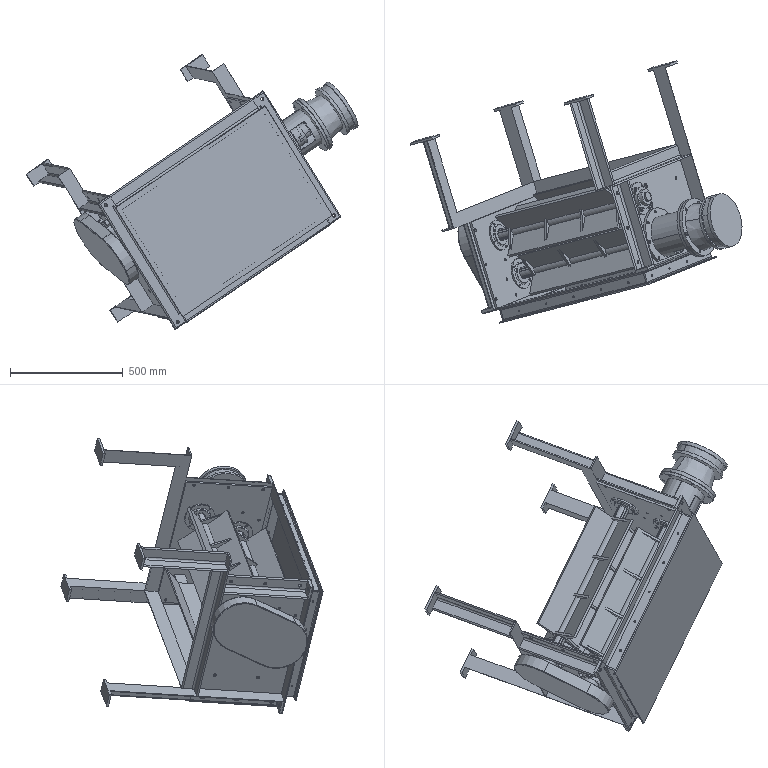Assembly | SolidWorks | mm | 25 component files | 27 solids | 1603 faces | box 1469.88 x 1161.19 x 1217.25 mm | volume 37875848 mm3 | plane 808 | cylinder 763 | cone 18 | torus 14 | commonest cylinder face diameters 12 x156 220 x86 14 x74 50 x48 7 x48 6 x41 8 x36 10 x32
Bill of materials:
CoarseCrusherGear | 2 |  | Thin disc-shaped spur gear with many straight teeth around the rim and a central round bore with one keyway notch.
CrusherFrame | 1 |  | Open box-shaped frame made of thin-walled straight profile members, with a rectangular frame at one end and long members running out to flanged or angled ends.
CrusherFrameBaffle | 1 |  | Long bent thin-sheet profile: a flat web with angled flanges along the long edges, forming an open channel or trough-like section.
CrusherFrameCoupling | 1 |  | Round hub part: a cylindrical spigot next to a larger-diameter flange section, a central through-bore, and evenly spaced radial slots cut into the flange face, leaving lug-like segments.
CrusherFrameSideCover | 1 |  | Rectangular thin-sheet tray or panel with shallow folded side walls and end flanges that carry U-shaped edge notches and small round holes.
CrusherFrameSpacer | 2 |  | Long straight bar with a square cross-section and a small hole in each end face. In one view the ends look like slightly offset square end pads with a hole.
CrusherFrameTopCover | 1 |  | Thin flat rectangular plate with narrow folded flanges along two opposite edges. The flanges carry a row of small holes.
CrusherGearCover | 1 |  | Obround (stadium-shaped) flat part of uniform thickness. One view looks like a shallow open tray with a thin perimeter wall around a recessed face.
CrusherMotorMount | 1 |  | Flanged cylindrical tube spool: a round tube with a bolt-hole flange at each end. One flange has a straight-cut edge, and a window opening is cut through the tube wall.
CutterAxisI | 1 |  | Rotor-like part: a central stepped round shaft carrying several flat radial blades along its length. Triangular gussets brace the blades against the shaft, and short shaft journals stick out at both ends.
CutterAxisII | 1 |  | Rotor-like part very similar to the previous one: a stepped round shaft with several radial flat blades, gusset plates along the blade roots, and shaft journals at both ends.
InnerDustCover | 4 |  | Flat circular flange ring with a large central bore, a raised concentric annular boss or spigot on one face, and four evenly spaced through-holes near the outer edge.
MotorCrusherFrameCoupling | 1 |  | Stepped, axially symmetric bushing-like part: a small cylindrical spigot with a through bore stands on a larger round collar, and the back face has a ring of radial lugs separated by notches (castellated).
UCFC208Bearing | 4 |  | Round flange plate with four through holes on a bolt circle, a raised annular step and a stepped central bore on the front, and cylindrical bosses on the back.
VerticalPlate | 2 |  | Thin flat rectangular plate with two large circular cutouts, each surrounded by a ring of small holes, plus small holes scattered across the plate and near its edges.
XLD-4CycloidReducer | 1 |  | Cylindrical housing-like body: one end has a mounting flange with a ring of small holes, the main body is stepped with a groove, the opposite end is a closed flat circular face, and a cylindrical shaft with a flat sticks out from the flange end.
Mates:
1. concentric | VerticalPlate-1 face at (-401.311, -161.07, -343.448) dir (-0.8088, -0.2094, -0.5495) r 50 | UCFC208Bearing-1 face at (-404.546, -161.908, -345.646) dir (0.8088, 0.2094, 0.5495) r 20
2. coincident | VerticalPlate-1 face at (-202.357, 27.392, -726.331) dir (-0.8088, -0.2094, -0.5495) | UCFC208Bearing-1 face at (-417.344, -204.256, -321.587) dir (0.8088, 0.2094, 0.5495)
3. concentric | VerticalPlate-1 face at (-304.381, -330.131, -421.698) dir (-0.8088, -0.2094, -0.5495) r 50 | UCFC208Bearing-2 face at (-307.616, -330.969, -423.896) dir (0.8088, 0.2094, 0.5495) r 43
4. coincident | VerticalPlate-1 face at (-202.357, 27.392, -726.331) dir (-0.8088, -0.2094, -0.5495) | UCFC208Bearing-2 face at (-338.104, -342.549, -385.524) dir (0.8088, 0.2094, 0.5495)
5. coincident | VerticalPlate-1 face at (-202.357, 27.392, -726.331) dir (-0.288, 0.9558, 0.05964) | VerticalPlate-2 face at (420.445, 188.642, -303.228) dir (-0.288, 0.9558, 0.05964)
6. distance | VerticalPlate-1 face at (-194.268, 29.487, -720.836) dir (0.8088, 0.2094, 0.5495) | VerticalPlate-2 face at (420.445, 188.642, -303.228) dir (-0.8088, -0.2094, -0.5495)
7. concentric | UCFC208Bearing-3 face at (216.638, -1.077, 76.358) dir (-0.8088, -0.2094, -0.5495) r 20 | VerticalPlate-2 face at (221.491, 0.1794, 79.655) dir (-0.8088, -0.2094, -0.5495) r 50
8. coincident | UCFC208Bearing-3 face at (229.436, 41.271, 52.299) dir (-0.8088, -0.2094, -0.5495) | VerticalPlate-2 face at (428.534, 190.736, -297.733) dir (0.8088, 0.2094, 0.5495)
9. concentric | UCFC208Bearing-4 face at (313.569, -170.138, -1.892) dir (-0.8088, -0.2094, -0.5495) r 20 | VerticalPlate-2 face at (318.422, -168.881, 1.405) dir (-0.8088, -0.2094, -0.5495) r 50
10. coincident | UCFC208Bearing-4 face at (289.844, -143.897, 33.949) dir (-0.8088, -0.2094, -0.5495) | VerticalPlate-2 face at (428.534, 190.736, -297.733) dir (0.8088, 0.2094, 0.5495)
11. concentric | UCFC208Bearing-4 face at (313.569, -170.138, -1.892) dir (-0.8088, -0.2094, -0.5495) r 20 | CutterAxisI-1 face at (360.885, -157.887, 30.253) dir (0.8088, 0.2094, 0.5495) r 20
12. distance | UCFC208Bearing-2 face at (-317.87, -335.098, -407.228) dir (0.8088, 0.2094, 0.5495) | CutterAxisI-1 face at (-309.175, -347.458, -412.586) dir (-0.8088, -0.2094, -0.5495)
13. concentric | CutterAxisI-1 face at (-391.33, -352.643, -480.767) dir (0.8088, 0.2094, 0.5495) r 17.5 | CoarseCrusherGear-1 face at (-391.33, -352.643, -480.767) dir (0.8088, 0.2094, 0.5495) r 17.5
14. coincident | CutterAxisI-1 face at (-391.33, -352.643, -480.767) dir (-0.8088, -0.2094, -0.5495) | CoarseCrusherGear-1 face at (-391.33, -352.643, -480.767) dir (-0.8088, -0.2094, -0.5495)
15. concentric | UCFC208Bearing-3 face at (216.638, -1.077, 76.358) dir (-0.8088, -0.2094, -0.5495) r 20 | CutterAxisII-1 face at (263.955, 11.174, 108.503) dir (0.8088, 0.2094, 0.5495) r 20
16. distance | UCFC208Bearing-3 face at (219.816, 15.36, 65.416) dir (-0.8088, -0.2094, -0.5495) | CutterAxisII-1 face at (218.978, 19.537, 62.328) dir (0.8088, 0.2094, 0.5495)
17. concentric | CoarseCrusherGear-2 face at (-488.261, -183.582, -402.518) dir (0.8088, 0.2094, 0.5495) r 17.5 | CutterAxisII-1 face at (-488.261, -183.582, -402.518) dir (0.8088, 0.2094, 0.5495) r 17.5
18. coincident | CoarseCrusherGear-2 face at (-488.261, -183.582, -402.518) dir (-0.8088, -0.2094, -0.5495) | CutterAxisII-1 face at (-488.261, -183.582, -402.518) dir (-0.8088, -0.2094, -0.5495)
19. concentric | CutterAxisI-1 face at (401.327, -147.416, 57.727) dir (-0.8088, -0.2094, -0.5495) r 17.5 | CrusherFrameCoupling-1 face at (413.46, -144.275, 65.97) dir (0.8088, 0.2094, 0.5495) r 29.5
20. coincident | CutterAxisI-1 face at (401.327, -147.416, 57.727) dir (0.8088, 0.2094, 0.5495) | CrusherFrameCoupling-1 face at (416.86, -196.379, 53.523) dir (0.8088, 0.2094, 0.5495)
21. concentric | UCFC208Bearing-1 face at (-404.546, -161.908, -345.646) dir (0.8088, 0.2094, 0.5495) r 20 | CutterAxisII-1 face at (263.955, 11.174, 108.503) dir (0.8088, 0.2094, 0.5495) r 20
22. coincident | VerticalPlate-2 face at (428.534, 190.736, -297.733) dir (0.8088, 0.2094, 0.5495) | CrusherFrame-1 face at (-54.541, 443.111, 317.164) dir (-0.8088, -0.2094, -0.5495)
23. coincident | VerticalPlate-2 face at (420.445, 188.642, -303.228) dir (-0.288, 0.9558, 0.05964) | CrusherFrame-1 face at (36.321, 32.782, 339.797) dir (0.288, -0.9558, -0.05964)
24. distance | VerticalPlate-2 face at (535.636, -193.669, -327.083) dir (0.5127, 0.2065, -0.8334) | CrusherFrame-1 face at (548.535, -178.92, -333.493) dir (0.5127, 0.2065, -0.8334)
25. coincident | CrusherFrame-1 face at (-183.839, -383.488, -759.141) dir (-0.5127, -0.2065, 0.8334) | CrusherFrameTopCover-1 face at (-109.81, -429.232, -724.931) dir (0.5127, 0.2065, -0.8334)
26. coincident | CrusherFrame-1 face at (-54.541, 443.111, 317.164) dir (-0.8088, -0.2094, -0.5495) | CrusherFrameTopCover-1 face at (250.147, -377.327, 181.345) dir (0.8088, 0.2094, 0.5495)
27. coincident | CrusherFrame-1 edge at (258.35, -374.023, 168.011) dir (0.5127, 0.2065, -0.8334) | CrusherFrameTopCover-1 face at (-396.92, -544.859, -258.242) dir (-0.288, 0.9558, 0.05964)
28. coincident | VerticalPlate-2 face at (420.445, 188.642, -303.228) dir (-0.8088, -0.2094, -0.5495) | CrusherFrameSpacer-1 face at (395.41, 71.384, -221.687) dir (0.8088, 0.2094, 0.5495)
29. distance | VerticalPlate-1 face at (-87.166, -354.919, -750.186) dir (0.5127, 0.2065, -0.8334) | CrusherFrameSpacer-1 face at (-223.051, -36.856, -634.986) dir (0.5127, 0.2065, -0.8334)
30. coincident | VerticalPlate-1 face at (-194.268, 29.487, -720.836) dir (0.8088, 0.2094, 0.5495) | CrusherFrameSpacer-2 face at (-186.22, -283.44, -613.423) dir (-0.8088, -0.2094, -0.5495)
31. coincident | CrusherFrameSpacer-1 face at (-223.051, -36.856, -634.986) dir (0.5127, 0.2065, -0.8334) | CrusherFrameSpacer-2 face at (-151.057, -275.8, -649.895) dir (0.5127, 0.2065, -0.8334)
32. distance | CrusherFrameSpacer-1 face at (372.339, 62.093, -184.186) dir (0.288, -0.9558, -0.05964) | CrusherFrameSpacer-2 face at (415.535, -81.274, -193.131) dir (-0.288, 0.9558, 0.05964)
33. distance | VerticalPlate-1 face at (-87.166, -354.919, -750.186) dir (0.288, -0.9558, -0.05964) | CrusherFrameSpacer-2 face at (-151.057, -275.8, -649.895) dir (0.288, -0.9558, -0.05964)
34. coincident | CrusherFrameSpacer-2 face at (415.535, -81.274, -193.131) dir (-0.5127, -0.2065, 0.8334) | CrusherFrameBaffle-1 face at (296.62, 94.005, -222.862) dir (0.5127, 0.2065, -0.8334)
35. coincident | CrusherFrameSpacer-1 edge at (349.851, 107.788, -186.699) dir (-0.8088, -0.2094, -0.5495) | CrusherFrameBaffle-1 edge at (296.62, 94.005, -222.862) dir (-0.8088, -0.2094, -0.5495)
36. coincident | CrusherFrame-1 face at (-322.682, 426.554, -712.259) dir (-0.8088, -0.2094, -0.5495) | CrusherFrameSideCover-1 face at (-87.785, -341.609, -765.268) dir (0.8088, 0.2094, 0.5495)
37. coincident | CrusherFrame-1 face at (-82.356, -342.264, -762.09) dir (0.5127, 0.2065, -0.8334) | CrusherFrameSideCover-1 face at (552.812, -175.752, -330.076) dir (-0.5127, -0.2065, 0.8334)
38. coincident | CrusherFrame-1 face at (-152.888, -377.453, -807.001) dir (0.288, -0.9558, -0.05964) | CrusherFrameSideCover-1 face at (-102.3, -366.863, -732.457) dir (-0.288, 0.9558, 0.05964)
39. concentric | CoarseCrusherGear-1 face at (-391.33, -352.643, -480.767) dir (0.8088, 0.2094, 0.5495) r 110 | CrusherGearCover-1 face at (-407.507, -356.831, -491.757) dir (0.8088, 0.2094, 0.5495) r 125
40. concentric | CoarseCrusherGear-2 face at (-488.261, -183.582, -402.518) dir (0.8088, 0.2094, 0.5495) r 110 | CrusherGearCover-1 face at (-504.437, -187.771, -413.507) dir (0.8088, 0.2094, 0.5495) r 127
41. distance | CoarseCrusherGear-2 face at (-488.261, -183.582, -402.518) dir (-0.8088, -0.2094, -0.5495) | CrusherGearCover-1 face at (-504.437, -187.771, -413.507) dir (0.8088, 0.2094, 0.5495)
42. coincident | VerticalPlate-2 face at (428.534, 190.736, -297.733) dir (0.8088, 0.2094, 0.5495) | CrusherMotorMount-1 face at (355.858, -293.132, -6.348) dir (-0.8088, -0.2094, -0.5495)
43. parallel | CrusherMotorMount-1 face at (307.144, -277.566, 95.825) dir (0.288, -0.9558, -0.05964) | CrusherFrame-1 face at (256.498, -303.86, 258.651) dir (-0.288, 0.9558, 0.05964)
44. coincident | CrusherFrameCoupling-1 face at (397.807, -177.847, 101.805) dir (-0.4148, 0.8655, 0.2808) | MotorCrusherFrameCoupling-1 face at (440.997, -130.686, 20.255) dir (0.4148, -0.8655, -0.2808)
45. coincident | CrusherFrameCoupling-1 face at (416.86, -196.379, 53.523) dir (0.8088, 0.2094, 0.5495) | MotorCrusherFrameCoupling-1 face at (391.95, -157.655, 75.433) dir (-0.8088, -0.2094, -0.5495)
46. concentric | UCFC208Bearing-3 face at (237.567, 44.927, 151.54) dir (-0.8088, -0.2094, -0.5495) r 7 | VerticalPlate-2 face at (195.61, 34.064, 123.037) dir (-0.8088, -0.2094, -0.5495) r 6
47. concentric | VerticalPlate-1 face at (-383.689, -109.666, -370.78) dir (-0.8088, -0.2094, -0.5495) r 6 | UCFC208Bearing-1 face at (-449.911, -126.811, -415.768) dir (0.8088, 0.2094, 0.5495) r 7
48. concentric | VerticalPlate-1 face at (-351.319, -346.708, -382.685) dir (0.8088, 0.2094, 0.5495) r 6 | UCFC208Bearing-2 face at (-393.276, -357.571, -411.189) dir (0.8088, 0.2094, 0.5495) r 7
49. concentric | MotorCrusherFrameCoupling-1 face at (401.327, -147.416, 57.727) dir (-0.8088, -0.2094, -0.5495) r 34.5 | XLD-4CycloidReducer-1 face at (413.46, -144.275, 65.97) dir (0.8088, 0.2094, 0.5495) r 22.5
50. coincident | MotorCrusherFrameCoupling-1 face at (413.46, -144.275, 65.97) dir (-0.8088, -0.2094, -0.5495) | XLD-4CycloidReducer-1 face at (413.46, -144.275, 65.97) dir (-0.8088, -0.2094, -0.5495)
51. concentric | CrusherFrameCoupling-1 face at (413.46, -144.275, 65.97) dir (0.8088, 0.2094, 0.5495) r 29.5 | MotorCrusherFrameCoupling-1 face at (401.327, -147.416, 57.727) dir (-0.8088, -0.2094, -0.5495) r 34.5
52. concentric | CutterAxisII-1 face at (263.955, 11.174, 108.503) dir (0.8088, 0.2094, 0.5495) r 25 | InnerDustCover-1 face at (-401.311, -161.07, -343.448) dir (-0.8088, -0.2094, -0.5495) r 26
53. coincident | VerticalPlate-1 face at (-194.268, 29.487, -720.836) dir (0.8088, 0.2094, 0.5495) | InnerDustCover-1 face at (-391.344, -147.53, -363.28) dir (-0.8088, -0.2094, -0.5495)
54. concentric | CutterAxisI-1 face at (360.885, -157.887, 30.253) dir (0.8088, 0.2094, 0.5495) r 25 | InnerDustCover-2 face at (-304.381, -330.131, -421.698) dir (-0.8088, -0.2094, -0.5495) r 26
55. coincident | VerticalPlate-1 face at (-194.268, 29.487, -720.836) dir (0.8088, 0.2094, 0.5495) | InnerDustCover-2 face at (-301.517, -307.668, -434.473) dir (-0.8088, -0.2094, -0.5495)
56. concentric | CutterAxisI-1 face at (360.885, -157.887, 30.253) dir (0.8088, 0.2094, 0.5495) r 25 | InnerDustCover-3 face at (310.333, -170.975, -4.09) dir (0.8088, 0.2094, 0.5495) r 26
57. coincident | VerticalPlate-2 face at (420.445, 188.642, -303.228) dir (-0.8088, -0.2094, -0.5495) | InnerDustCover-3 face at (297.45, -151.583, 7.484) dir (0.8088, 0.2094, 0.5495)
58. concentric | CutterAxisII-1 face at (263.955, 11.174, 108.503) dir (0.8088, 0.2094, 0.5495) r 25 | InnerDustCover-4 face at (213.403, -1.915, 74.16) dir (0.8088, 0.2094, 0.5495) r 26
59. coincident | VerticalPlate-2 face at (420.445, 188.642, -303.228) dir (-0.8088, -0.2094, -0.5495) | InnerDustCover-4 face at (199.378, 14.628, 88.5) dir (0.8088, 0.2094, 0.5495)